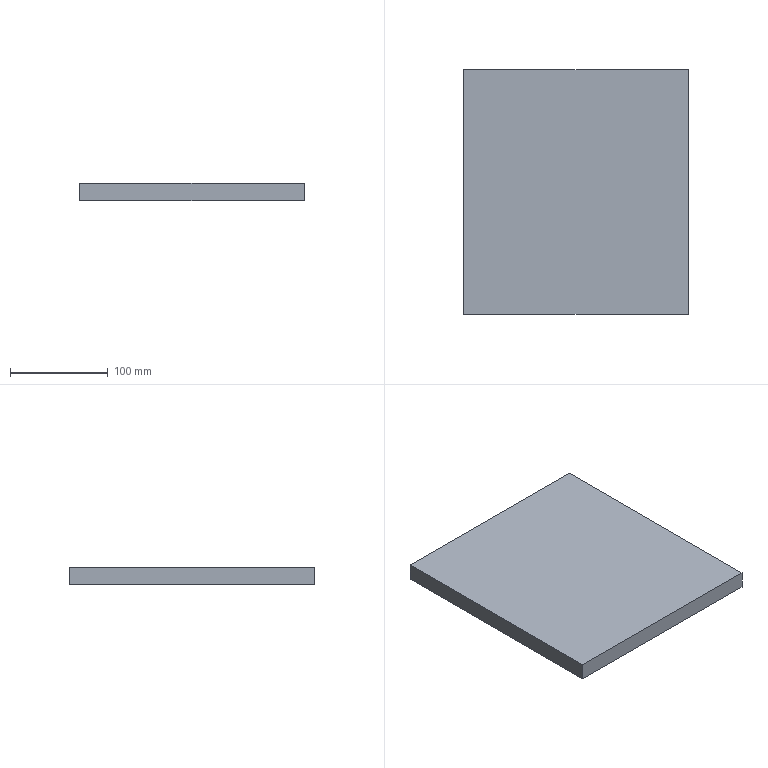Component | NX | WORKPIECE | 1 solid | 6 faces | box 230 x 250 x 17.7 mm | volume 1017750 mm3 | plane 6
STEP:
#1=CARTESIAN_POINT('',(0.,0.,0.));
#2=DIRECTION('',(0.,0.,1.));
#3=DIRECTION('',(1.,0.,0.));
#4=AXIS2_PLACEMENT_3D('',#1,#2,#3);
#5=CARTESIAN_POINT('',(-115.,125.,87.5));
#6=VERTEX_POINT('',#5);
#7=CARTESIAN_POINT('',(-115.,-125.,87.5));
#8=VERTEX_POINT('',#7);
#9=CARTESIAN_POINT('',(-115.,125.,87.5));
#10=DIRECTION('',(0.,-1.,0.));
#11=VECTOR('',#10,1.);
#12=LINE('',#9,#11);
#13=CARTESIAN_POINT('',(-115.,125.,105.2));
#14=DIRECTION('',(1.,0.,0.));
#15=DIRECTION('',(0.,0.,-1.));
#16=AXIS2_PLACEMENT_3D('',#13,#14,#15);
#17=PLANE('',#16);
#18=CARTESIAN_POINT('',(17.7,0.));
#19=DIRECTION('',(0.,-1.));
#20=VECTOR('',#19,1.);
#21=LINE('',#18,#20);
#22=(GEOMETRIC_REPRESENTATION_CONTEXT(2)PARAMETRIC_REPRESENTATION_CONTEXT()REPRESENTATION_CONTEXT('',''));
#23=DEFINITIONAL_REPRESENTATION('',(#21),#22);
#24=PCURVE('',#17,#23);
#25=CARTESIAN_POINT('',(-0.,-0.,87.5));
#26=DIRECTION('',(0.,0.,1.));
#27=DIRECTION('',(1.,0.,0.));
#28=AXIS2_PLACEMENT_3D('',#25,#26,#27);
#29=PLANE('',#28);
#30=CARTESIAN_POINT('',(-115.,125.));
#31=DIRECTION('',(0.,-1.));
#32=VECTOR('',#31,1.);
#33=LINE('',#30,#32);
#34=(GEOMETRIC_REPRESENTATION_CONTEXT(2)PARAMETRIC_REPRESENTATION_CONTEXT()REPRESENTATION_CONTEXT('',''));
#35=DEFINITIONAL_REPRESENTATION('',(#33),#34);
#36=PCURVE('',#29,#35);
#37=SURFACE_CURVE('',#12,(#24,#36),.PCURVE_S1.);
#38=EDGE_CURVE('',#6,#8,#37,.T.);
#39=ORIENTED_EDGE('',*,*,#38,.T.);
#40=CARTESIAN_POINT('',(-115.,-125.,105.2));
#41=VERTEX_POINT('',#40);
#42=CARTESIAN_POINT('',(-115.,-125.,105.2));
#43=DIRECTION('',(0.,0.,-1.));
#44=VECTOR('',#43,1.);
#45=LINE('',#42,#44);
#46=CARTESIAN_POINT('',(0.,-250.));
#47=DIRECTION('',(1.,0.));
#48=VECTOR('',#47,1.);
#49=LINE('',#46,#48);
#50=(GEOMETRIC_REPRESENTATION_CONTEXT(2)PARAMETRIC_REPRESENTATION_CONTEXT()REPRESENTATION_CONTEXT('',''));
#51=DEFINITIONAL_REPRESENTATION('',(#49),#50);
#52=PCURVE('',#17,#51);
#53=CARTESIAN_POINT('',(-115.,-125.,105.2));
#54=DIRECTION('',(0.,1.,0.));
#55=DIRECTION('',(0.,0.,1.));
#56=AXIS2_PLACEMENT_3D('',#53,#54,#55);
#57=PLANE('',#56);
#58=CARTESIAN_POINT('',(0.,0.));
#59=DIRECTION('',(-1.,0.));
#60=VECTOR('',#59,1.);
#61=LINE('',#58,#60);
#62=(GEOMETRIC_REPRESENTATION_CONTEXT(2)PARAMETRIC_REPRESENTATION_CONTEXT()REPRESENTATION_CONTEXT('',''));
#63=DEFINITIONAL_REPRESENTATION('',(#61),#62);
#64=PCURVE('',#57,#63);
#65=SURFACE_CURVE('',#45,(#52,#64),.PCURVE_S1.);
#66=EDGE_CURVE('',#41,#8,#65,.T.);
#67=ORIENTED_EDGE('',*,*,#66,.F.);
#68=CARTESIAN_POINT('',(-115.,125.,105.2));
#69=VERTEX_POINT('',#68);
#70=CARTESIAN_POINT('',(-115.,125.,105.2));
#71=DIRECTION('',(0.,-1.,0.));
#72=VECTOR('',#71,1.);
#73=LINE('',#70,#72);
#74=CARTESIAN_POINT('',(0.,0.));
#75=DIRECTION('',(0.,-1.));
#76=VECTOR('',#75,1.);
#77=LINE('',#74,#76);
#78=(GEOMETRIC_REPRESENTATION_CONTEXT(2)PARAMETRIC_REPRESENTATION_CONTEXT()REPRESENTATION_CONTEXT('',''));
#79=DEFINITIONAL_REPRESENTATION('',(#77),#78);
#80=PCURVE('',#17,#79);
#81=CARTESIAN_POINT('',(-0.,-0.,105.2));
#82=DIRECTION('',(0.,0.,1.));
#83=DIRECTION('',(1.,0.,0.));
#84=AXIS2_PLACEMENT_3D('',#81,#82,#83);
#85=PLANE('',#84);
#86=CARTESIAN_POINT('',(-115.,125.));
#87=DIRECTION('',(0.,-1.));
#88=VECTOR('',#87,1.);
#89=LINE('',#86,#88);
#90=(GEOMETRIC_REPRESENTATION_CONTEXT(2)PARAMETRIC_REPRESENTATION_CONTEXT()REPRESENTATION_CONTEXT('',''));
#91=DEFINITIONAL_REPRESENTATION('',(#89),#90);
#92=PCURVE('',#85,#91);
#93=SURFACE_CURVE('',#73,(#80,#92),.PCURVE_S1.);
#94=EDGE_CURVE('',#69,#41,#93,.T.);
#95=ORIENTED_EDGE('',*,*,#94,.F.);
#96=CARTESIAN_POINT('',(-115.,125.,105.2));
#97=DIRECTION('',(0.,0.,-1.));
#98=VECTOR('',#97,1.);
#99=LINE('',#96,#98);
#100=CARTESIAN_POINT('',(0.,0.));
#101=DIRECTION('',(1.,0.));
#102=VECTOR('',#101,1.);
#103=LINE('',#100,#102);
#104=(GEOMETRIC_REPRESENTATION_CONTEXT(2)PARAMETRIC_REPRESENTATION_CONTEXT()REPRESENTATION_CONTEXT('',''));
#105=DEFINITIONAL_REPRESENTATION('',(#103),#104);
#106=PCURVE('',#17,#105);
#107=CARTESIAN_POINT('',(115.,125.,105.2));
#108=DIRECTION('',(0.,-1.,0.));
#109=DIRECTION('',(0.,0.,-1.));
#110=AXIS2_PLACEMENT_3D('',#107,#108,#109);
#111=PLANE('',#110);
#112=CARTESIAN_POINT('',(0.,-230.));
#113=DIRECTION('',(1.,0.));
#114=VECTOR('',#113,1.);
#115=LINE('',#112,#114);
#116=(GEOMETRIC_REPRESENTATION_CONTEXT(2)PARAMETRIC_REPRESENTATION_CONTEXT()REPRESENTATION_CONTEXT('',''));
#117=DEFINITIONAL_REPRESENTATION('',(#115),#116);
#118=PCURVE('',#111,#117);
#119=SURFACE_CURVE('',#99,(#106,#118),.PCURVE_S1.);
#120=EDGE_CURVE('',#69,#6,#119,.T.);
#121=ORIENTED_EDGE('',*,*,#120,.T.);
#122=EDGE_LOOP('',(#39,#67,#95,#121));
#123=FACE_BOUND('',#122,.T.);
#124=ADVANCED_FACE('',(#123),#17,.F.);
#125=CARTESIAN_POINT('',(115.,-125.,87.5));
#126=VERTEX_POINT('',#125);
#127=CARTESIAN_POINT('',(-115.,-125.,87.5));
#128=DIRECTION('',(1.,0.,0.));
#129=VECTOR('',#128,1.);
#130=LINE('',#127,#129);
#131=CARTESIAN_POINT('',(-17.7,0.));
#132=DIRECTION('',(0.,1.));
#133=VECTOR('',#132,1.);
#134=LINE('',#131,#133);
#135=(GEOMETRIC_REPRESENTATION_CONTEXT(2)PARAMETRIC_REPRESENTATION_CONTEXT()REPRESENTATION_CONTEXT('',''));
#136=DEFINITIONAL_REPRESENTATION('',(#134),#135);
#137=PCURVE('',#57,#136);
#138=CARTESIAN_POINT('',(-115.,-125.));
#139=DIRECTION('',(1.,0.));
#140=VECTOR('',#139,1.);
#141=LINE('',#138,#140);
#142=(GEOMETRIC_REPRESENTATION_CONTEXT(2)PARAMETRIC_REPRESENTATION_CONTEXT()REPRESENTATION_CONTEXT('',''));
#143=DEFINITIONAL_REPRESENTATION('',(#141),#142);
#144=PCURVE('',#29,#143);
#145=SURFACE_CURVE('',#130,(#137,#144),.PCURVE_S1.);
#146=EDGE_CURVE('',#8,#126,#145,.T.);
#147=ORIENTED_EDGE('',*,*,#146,.T.);
#148=CARTESIAN_POINT('',(115.,-125.,105.2));
#149=VERTEX_POINT('',#148);
#150=CARTESIAN_POINT('',(115.,-125.,105.2));
#151=DIRECTION('',(0.,0.,-1.));
#152=VECTOR('',#151,1.);
#153=LINE('',#150,#152);
#154=CARTESIAN_POINT('',(0.,230.));
#155=DIRECTION('',(-1.,0.));
#156=VECTOR('',#155,1.);
#157=LINE('',#154,#156);
#158=(GEOMETRIC_REPRESENTATION_CONTEXT(2)PARAMETRIC_REPRESENTATION_CONTEXT()REPRESENTATION_CONTEXT('',''));
#159=DEFINITIONAL_REPRESENTATION('',(#157),#158);
#160=PCURVE('',#57,#159);
#161=CARTESIAN_POINT('',(115.,-125.,105.2));
#162=DIRECTION('',(-1.,0.,0.));
#163=DIRECTION('',(0.,0.,1.));
#164=AXIS2_PLACEMENT_3D('',#161,#162,#163);
#165=PLANE('',#164);
#166=CARTESIAN_POINT('',(0.,0.));
#167=DIRECTION('',(-1.,0.));
#168=VECTOR('',#167,1.);
#169=LINE('',#166,#168);
#170=(GEOMETRIC_REPRESENTATION_CONTEXT(2)PARAMETRIC_REPRESENTATION_CONTEXT()REPRESENTATION_CONTEXT('',''));
#171=DEFINITIONAL_REPRESENTATION('',(#169),#170);
#172=PCURVE('',#165,#171);
#173=SURFACE_CURVE('',#153,(#160,#172),.PCURVE_S1.);
#174=EDGE_CURVE('',#149,#126,#173,.T.);
#175=ORIENTED_EDGE('',*,*,#174,.F.);
#176=CARTESIAN_POINT('',(-115.,-125.,105.2));
#177=DIRECTION('',(1.,0.,0.));
#178=VECTOR('',#177,1.);
#179=LINE('',#176,#178);
#180=CARTESIAN_POINT('',(0.,0.));
#181=DIRECTION('',(0.,1.));
#182=VECTOR('',#181,1.);
#183=LINE('',#180,#182);
#184=(GEOMETRIC_REPRESENTATION_CONTEXT(2)PARAMETRIC_REPRESENTATION_CONTEXT()REPRESENTATION_CONTEXT('',''));
#185=DEFINITIONAL_REPRESENTATION('',(#183),#184);
#186=PCURVE('',#57,#185);
#187=CARTESIAN_POINT('',(-115.,-125.));
#188=DIRECTION('',(1.,0.));
#189=VECTOR('',#188,1.);
#190=LINE('',#187,#189);
#191=(GEOMETRIC_REPRESENTATION_CONTEXT(2)PARAMETRIC_REPRESENTATION_CONTEXT()REPRESENTATION_CONTEXT('',''));
#192=DEFINITIONAL_REPRESENTATION('',(#190),#191);
#193=PCURVE('',#85,#192);
#194=SURFACE_CURVE('',#179,(#186,#193),.PCURVE_S1.);
#195=EDGE_CURVE('',#41,#149,#194,.T.);
#196=ORIENTED_EDGE('',*,*,#195,.F.);
#197=ORIENTED_EDGE('',*,*,#66,.T.);
#198=EDGE_LOOP('',(#147,#175,#196,#197));
#199=FACE_BOUND('',#198,.T.);
#200=ADVANCED_FACE('',(#199),#57,.F.);
#201=CARTESIAN_POINT('',(115.,125.,87.5));
#202=VERTEX_POINT('',#201);
#203=CARTESIAN_POINT('',(115.,-125.,87.5));
#204=DIRECTION('',(0.,1.,0.));
#205=VECTOR('',#204,1.);
#206=LINE('',#203,#205);
#207=CARTESIAN_POINT('',(-17.7,0.));
#208=DIRECTION('',(0.,1.));
#209=VECTOR('',#208,1.);
#210=LINE('',#207,#209);
#211=(GEOMETRIC_REPRESENTATION_CONTEXT(2)PARAMETRIC_REPRESENTATION_CONTEXT()REPRESENTATION_CONTEXT('',''));
#212=DEFINITIONAL_REPRESENTATION('',(#210),#211);
#213=PCURVE('',#165,#212);
#214=CARTESIAN_POINT('',(115.,-125.));
#215=DIRECTION('',(0.,1.));
#216=VECTOR('',#215,1.);
#217=LINE('',#214,#216);
#218=(GEOMETRIC_REPRESENTATION_CONTEXT(2)PARAMETRIC_REPRESENTATION_CONTEXT()REPRESENTATION_CONTEXT('',''));
#219=DEFINITIONAL_REPRESENTATION('',(#217),#218);
#220=PCURVE('',#29,#219);
#221=SURFACE_CURVE('',#206,(#213,#220),.PCURVE_S1.);
#222=EDGE_CURVE('',#126,#202,#221,.T.);
#223=ORIENTED_EDGE('',*,*,#222,.T.);
#224=CARTESIAN_POINT('',(115.,125.,105.2));
#225=VERTEX_POINT('',#224);
#226=CARTESIAN_POINT('',(115.,125.,105.2));
#227=DIRECTION('',(0.,0.,-1.));
#228=VECTOR('',#227,1.);
#229=LINE('',#226,#228);
#230=CARTESIAN_POINT('',(0.,250.));
#231=DIRECTION('',(-1.,0.));
#232=VECTOR('',#231,1.);
#233=LINE('',#230,#232);
#234=(GEOMETRIC_REPRESENTATION_CONTEXT(2)PARAMETRIC_REPRESENTATION_CONTEXT()REPRESENTATION_CONTEXT('',''));
#235=DEFINITIONAL_REPRESENTATION('',(#233),#234);
#236=PCURVE('',#165,#235);
#237=CARTESIAN_POINT('',(0.,0.));
#238=DIRECTION('',(1.,0.));
#239=VECTOR('',#238,1.);
#240=LINE('',#237,#239);
#241=(GEOMETRIC_REPRESENTATION_CONTEXT(2)PARAMETRIC_REPRESENTATION_CONTEXT()REPRESENTATION_CONTEXT('',''));
#242=DEFINITIONAL_REPRESENTATION('',(#240),#241);
#243=PCURVE('',#111,#242);
#244=SURFACE_CURVE('',#229,(#236,#243),.PCURVE_S1.);
#245=EDGE_CURVE('',#225,#202,#244,.T.);
#246=ORIENTED_EDGE('',*,*,#245,.F.);
#247=CARTESIAN_POINT('',(115.,-125.,105.2));
#248=DIRECTION('',(0.,1.,0.));
#249=VECTOR('',#248,1.);
#250=LINE('',#247,#249);
#251=CARTESIAN_POINT('',(0.,0.));
#252=DIRECTION('',(0.,1.));
#253=VECTOR('',#252,1.);
#254=LINE('',#251,#253);
#255=(GEOMETRIC_REPRESENTATION_CONTEXT(2)PARAMETRIC_REPRESENTATION_CONTEXT()REPRESENTATION_CONTEXT('',''));
#256=DEFINITIONAL_REPRESENTATION('',(#254),#255);
#257=PCURVE('',#165,#256);
#258=CARTESIAN_POINT('',(115.,-125.));
#259=DIRECTION('',(0.,1.));
#260=VECTOR('',#259,1.);
#261=LINE('',#258,#260);
#262=(GEOMETRIC_REPRESENTATION_CONTEXT(2)PARAMETRIC_REPRESENTATION_CONTEXT()REPRESENTATION_CONTEXT('',''));
#263=DEFINITIONAL_REPRESENTATION('',(#261),#262);
#264=PCURVE('',#85,#263);
#265=SURFACE_CURVE('',#250,(#257,#264),.PCURVE_S1.);
#266=EDGE_CURVE('',#149,#225,#265,.T.);
#267=ORIENTED_EDGE('',*,*,#266,.F.);
#268=ORIENTED_EDGE('',*,*,#174,.T.);
#269=EDGE_LOOP('',(#223,#246,#267,#268));
#270=FACE_BOUND('',#269,.T.);
#271=ADVANCED_FACE('',(#270),#165,.F.);
#272=CARTESIAN_POINT('',(115.,125.,87.5));
#273=DIRECTION('',(-1.,0.,0.));
#274=VECTOR('',#273,1.);
#275=LINE('',#272,#274);
#276=CARTESIAN_POINT('',(17.7,0.));
#277=DIRECTION('',(0.,-1.));
#278=VECTOR('',#277,1.);
#279=LINE('',#276,#278);
#280=(GEOMETRIC_REPRESENTATION_CONTEXT(2)PARAMETRIC_REPRESENTATION_CONTEXT()REPRESENTATION_CONTEXT('',''));
#281=DEFINITIONAL_REPRESENTATION('',(#279),#280);
#282=PCURVE('',#111,#281);
#283=CARTESIAN_POINT('',(115.,125.));
#284=DIRECTION('',(-1.,0.));
#285=VECTOR('',#284,1.);
#286=LINE('',#283,#285);
#287=(GEOMETRIC_REPRESENTATION_CONTEXT(2)PARAMETRIC_REPRESENTATION_CONTEXT()REPRESENTATION_CONTEXT('',''));
#288=DEFINITIONAL_REPRESENTATION('',(#286),#287);
#289=PCURVE('',#29,#288);
#290=SURFACE_CURVE('',#275,(#282,#289),.PCURVE_S1.);
#291=EDGE_CURVE('',#202,#6,#290,.T.);
#292=ORIENTED_EDGE('',*,*,#291,.T.);
#293=ORIENTED_EDGE('',*,*,#120,.F.);
#294=CARTESIAN_POINT('',(115.,125.,105.2));
#295=DIRECTION('',(-1.,0.,0.));
#296=VECTOR('',#295,1.);
#297=LINE('',#294,#296);
#298=CARTESIAN_POINT('',(0.,0.));
#299=DIRECTION('',(0.,-1.));
#300=VECTOR('',#299,1.);
#301=LINE('',#298,#300);
#302=(GEOMETRIC_REPRESENTATION_CONTEXT(2)PARAMETRIC_REPRESENTATION_CONTEXT()REPRESENTATION_CONTEXT('',''));
#303=DEFINITIONAL_REPRESENTATION('',(#301),#302);
#304=PCURVE('',#111,#303);
#305=CARTESIAN_POINT('',(115.,125.));
#306=DIRECTION('',(-1.,0.));
#307=VECTOR('',#306,1.);
#308=LINE('',#305,#307);
#309=(GEOMETRIC_REPRESENTATION_CONTEXT(2)PARAMETRIC_REPRESENTATION_CONTEXT()REPRESENTATION_CONTEXT('',''));
#310=DEFINITIONAL_REPRESENTATION('',(#308),#309);
#311=PCURVE('',#85,#310);
#312=SURFACE_CURVE('',#297,(#304,#311),.PCURVE_S1.);
#313=EDGE_CURVE('',#225,#69,#312,.T.);
#314=ORIENTED_EDGE('',*,*,#313,.F.);
#315=ORIENTED_EDGE('',*,*,#245,.T.);
#316=EDGE_LOOP('',(#292,#293,#314,#315));
#317=FACE_BOUND('',#316,.T.);
#318=ADVANCED_FACE('',(#317),#111,.F.);
#319=ORIENTED_EDGE('',*,*,#94,.T.);
#320=ORIENTED_EDGE('',*,*,#195,.T.);
#321=ORIENTED_EDGE('',*,*,#266,.T.);
#322=ORIENTED_EDGE('',*,*,#313,.T.);
#323=EDGE_LOOP('',(#319,#320,#321,#322));
#324=FACE_BOUND('',#323,.T.);
#325=ADVANCED_FACE('',(#324),#85,.T.);
#326=ORIENTED_EDGE('',*,*,#38,.F.);
#327=ORIENTED_EDGE('',*,*,#291,.F.);
#328=ORIENTED_EDGE('',*,*,#222,.F.);
#329=ORIENTED_EDGE('',*,*,#146,.F.);
#330=EDGE_LOOP('',(#326,#327,#328,#329));
#331=FACE_BOUND('',#330,.T.);
#332=ADVANCED_FACE('',(#331),#29,.F.);
#333=CLOSED_SHELL('',(#124,#200,#271,#318,#325,#332));
#334=MANIFOLD_SOLID_BREP('',#333);
#335=(LENGTH_UNIT()NAMED_UNIT(*)SI_UNIT(.MILLI.,.METRE.));
#336=UNCERTAINTY_MEASURE_WITH_UNIT(LENGTH_MEASURE(0.0000001),#335,'','');
#337=(NAMED_UNIT(*)PLANE_ANGLE_UNIT()SI_UNIT($,.RADIAN.));
#338=(NAMED_UNIT(*)SI_UNIT($,.STERADIAN.)SOLID_ANGLE_UNIT());
#339=(GEOMETRIC_REPRESENTATION_CONTEXT(3)GLOBAL_UNCERTAINTY_ASSIGNED_CONTEXT((#336))GLOBAL_UNIT_ASSIGNED_CONTEXT((#335,#337,#338))REPRESENTATION_CONTEXT('',''));
#340=ADVANCED_BREP_SHAPE_REPRESENTATION('',(#4,#334),#339);